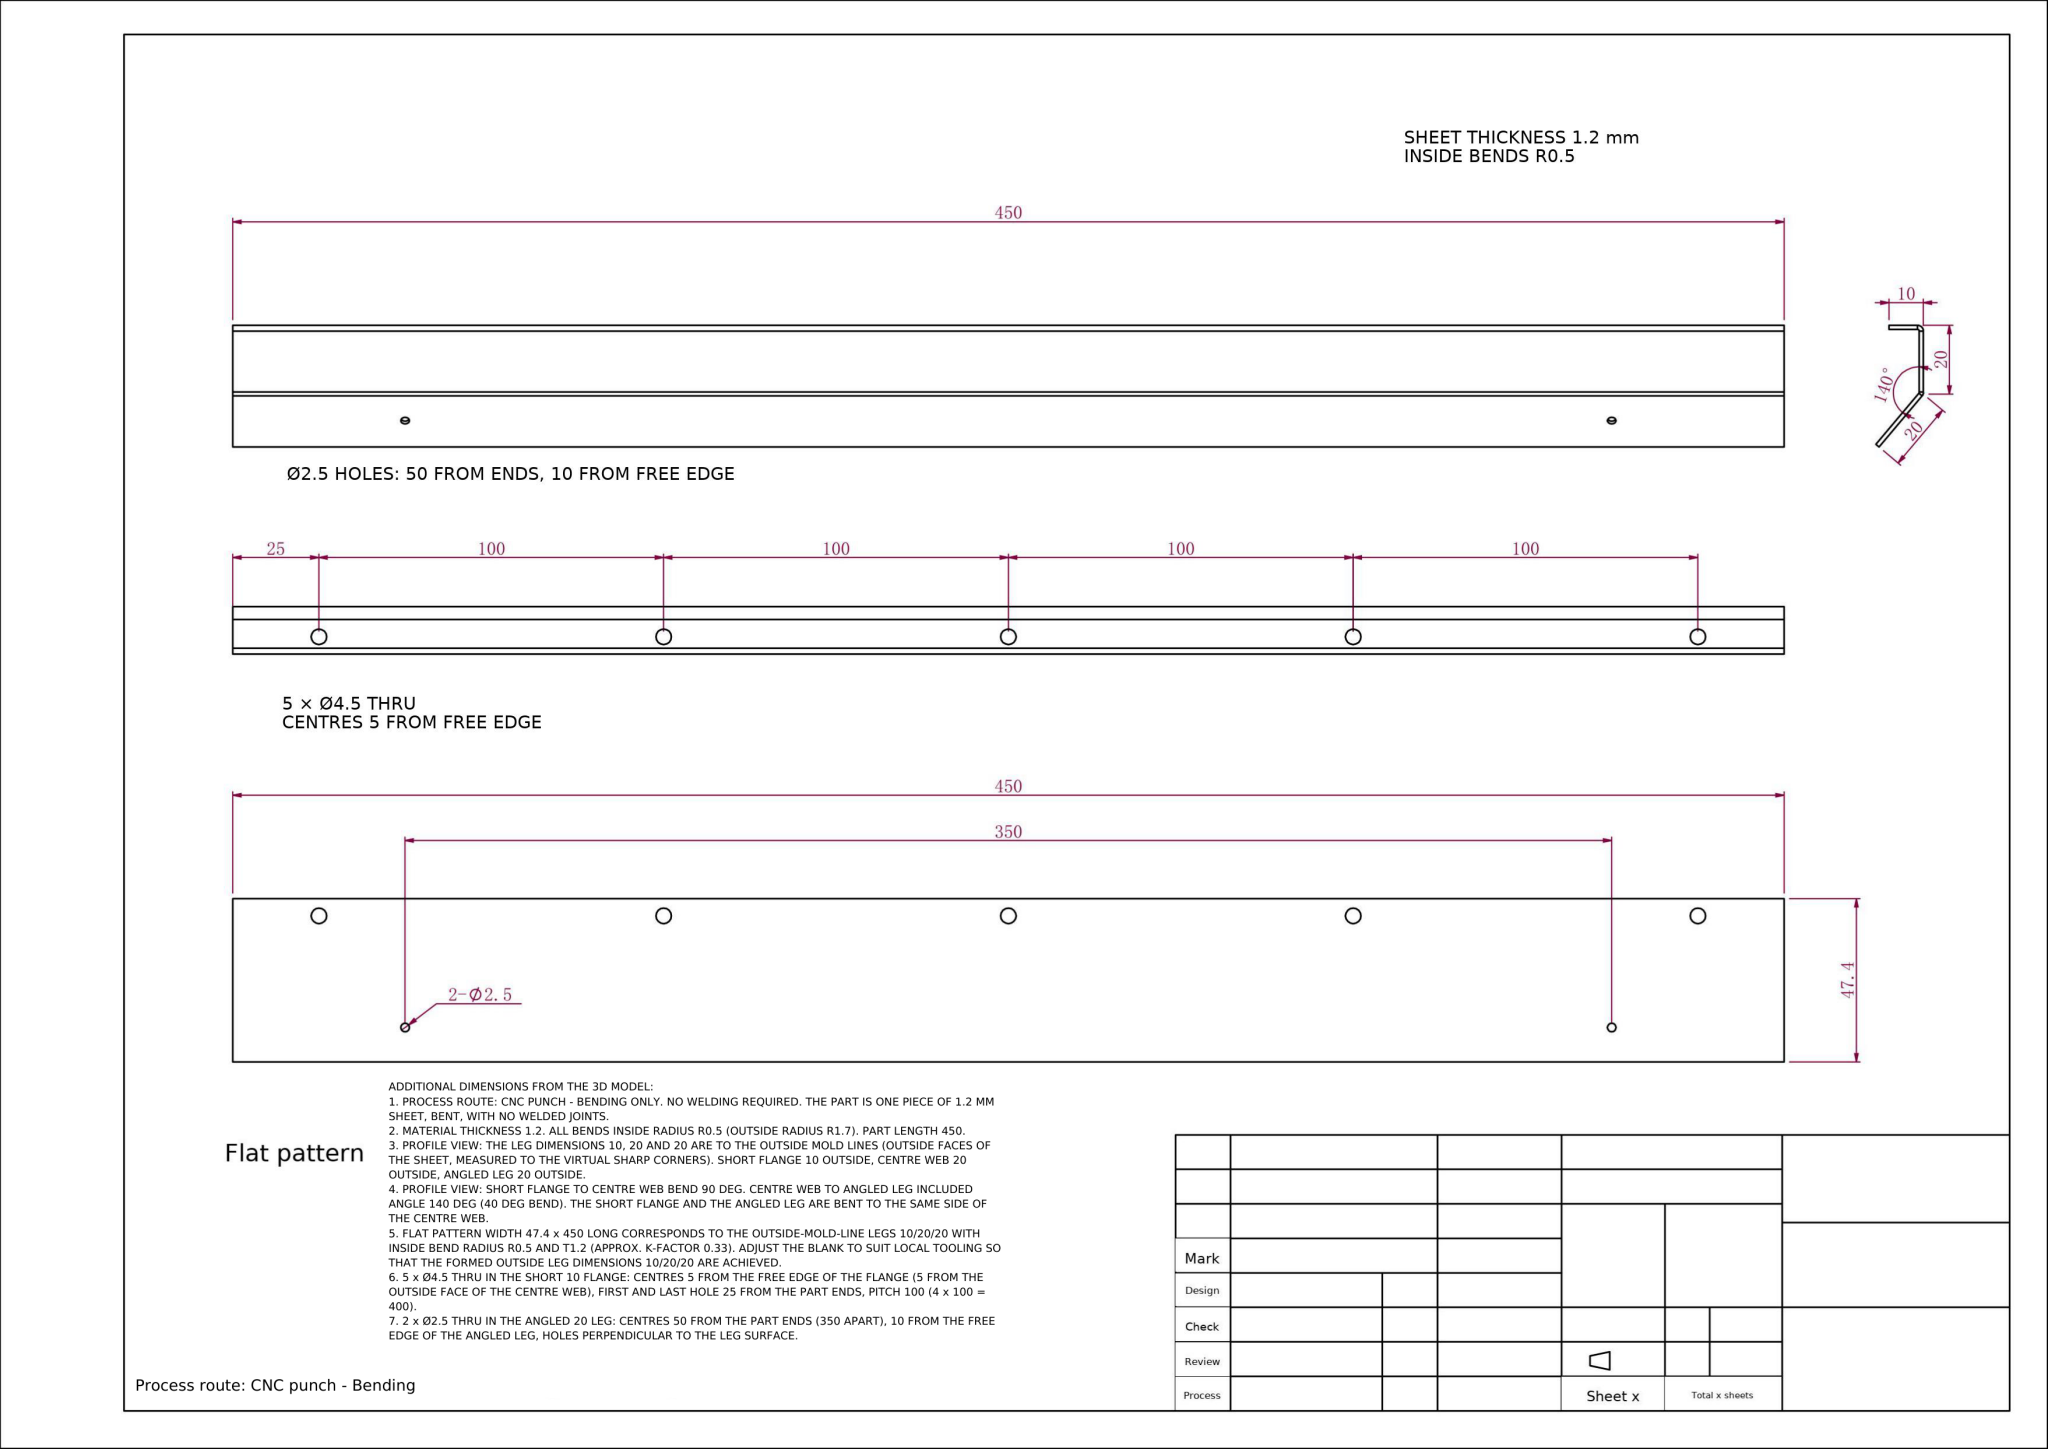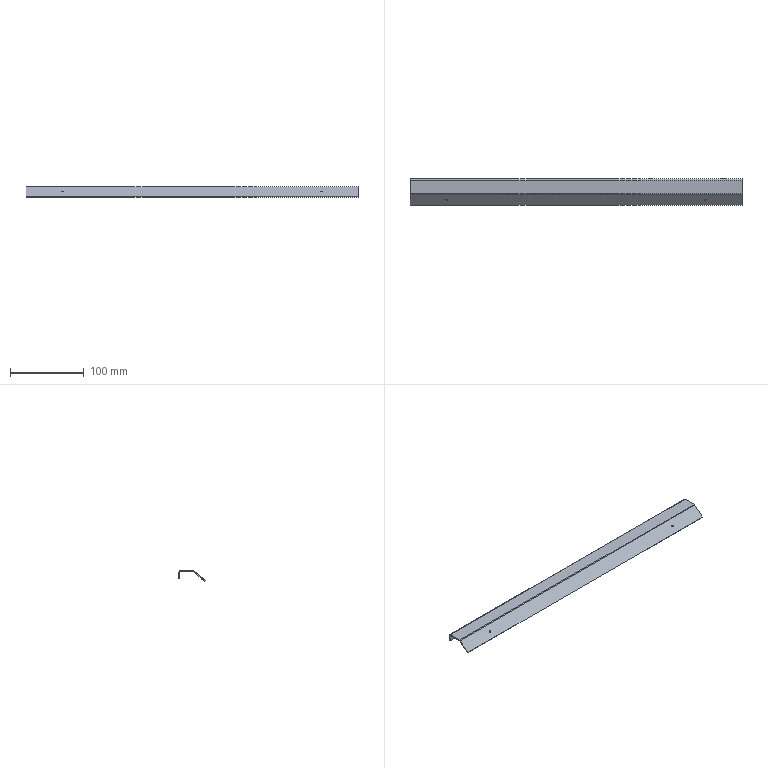Part | NX | mm | Five-Hole U-Channel Rail Beam | 1 solid | 36 faces | box 450 x 35.32 x 13.78 mm | volume 25736 mm3 | cylinder 18 | plane 18 | commonest cylinder face diameters 4.5 x10 2.5 x4 3.4 x2 1 x2